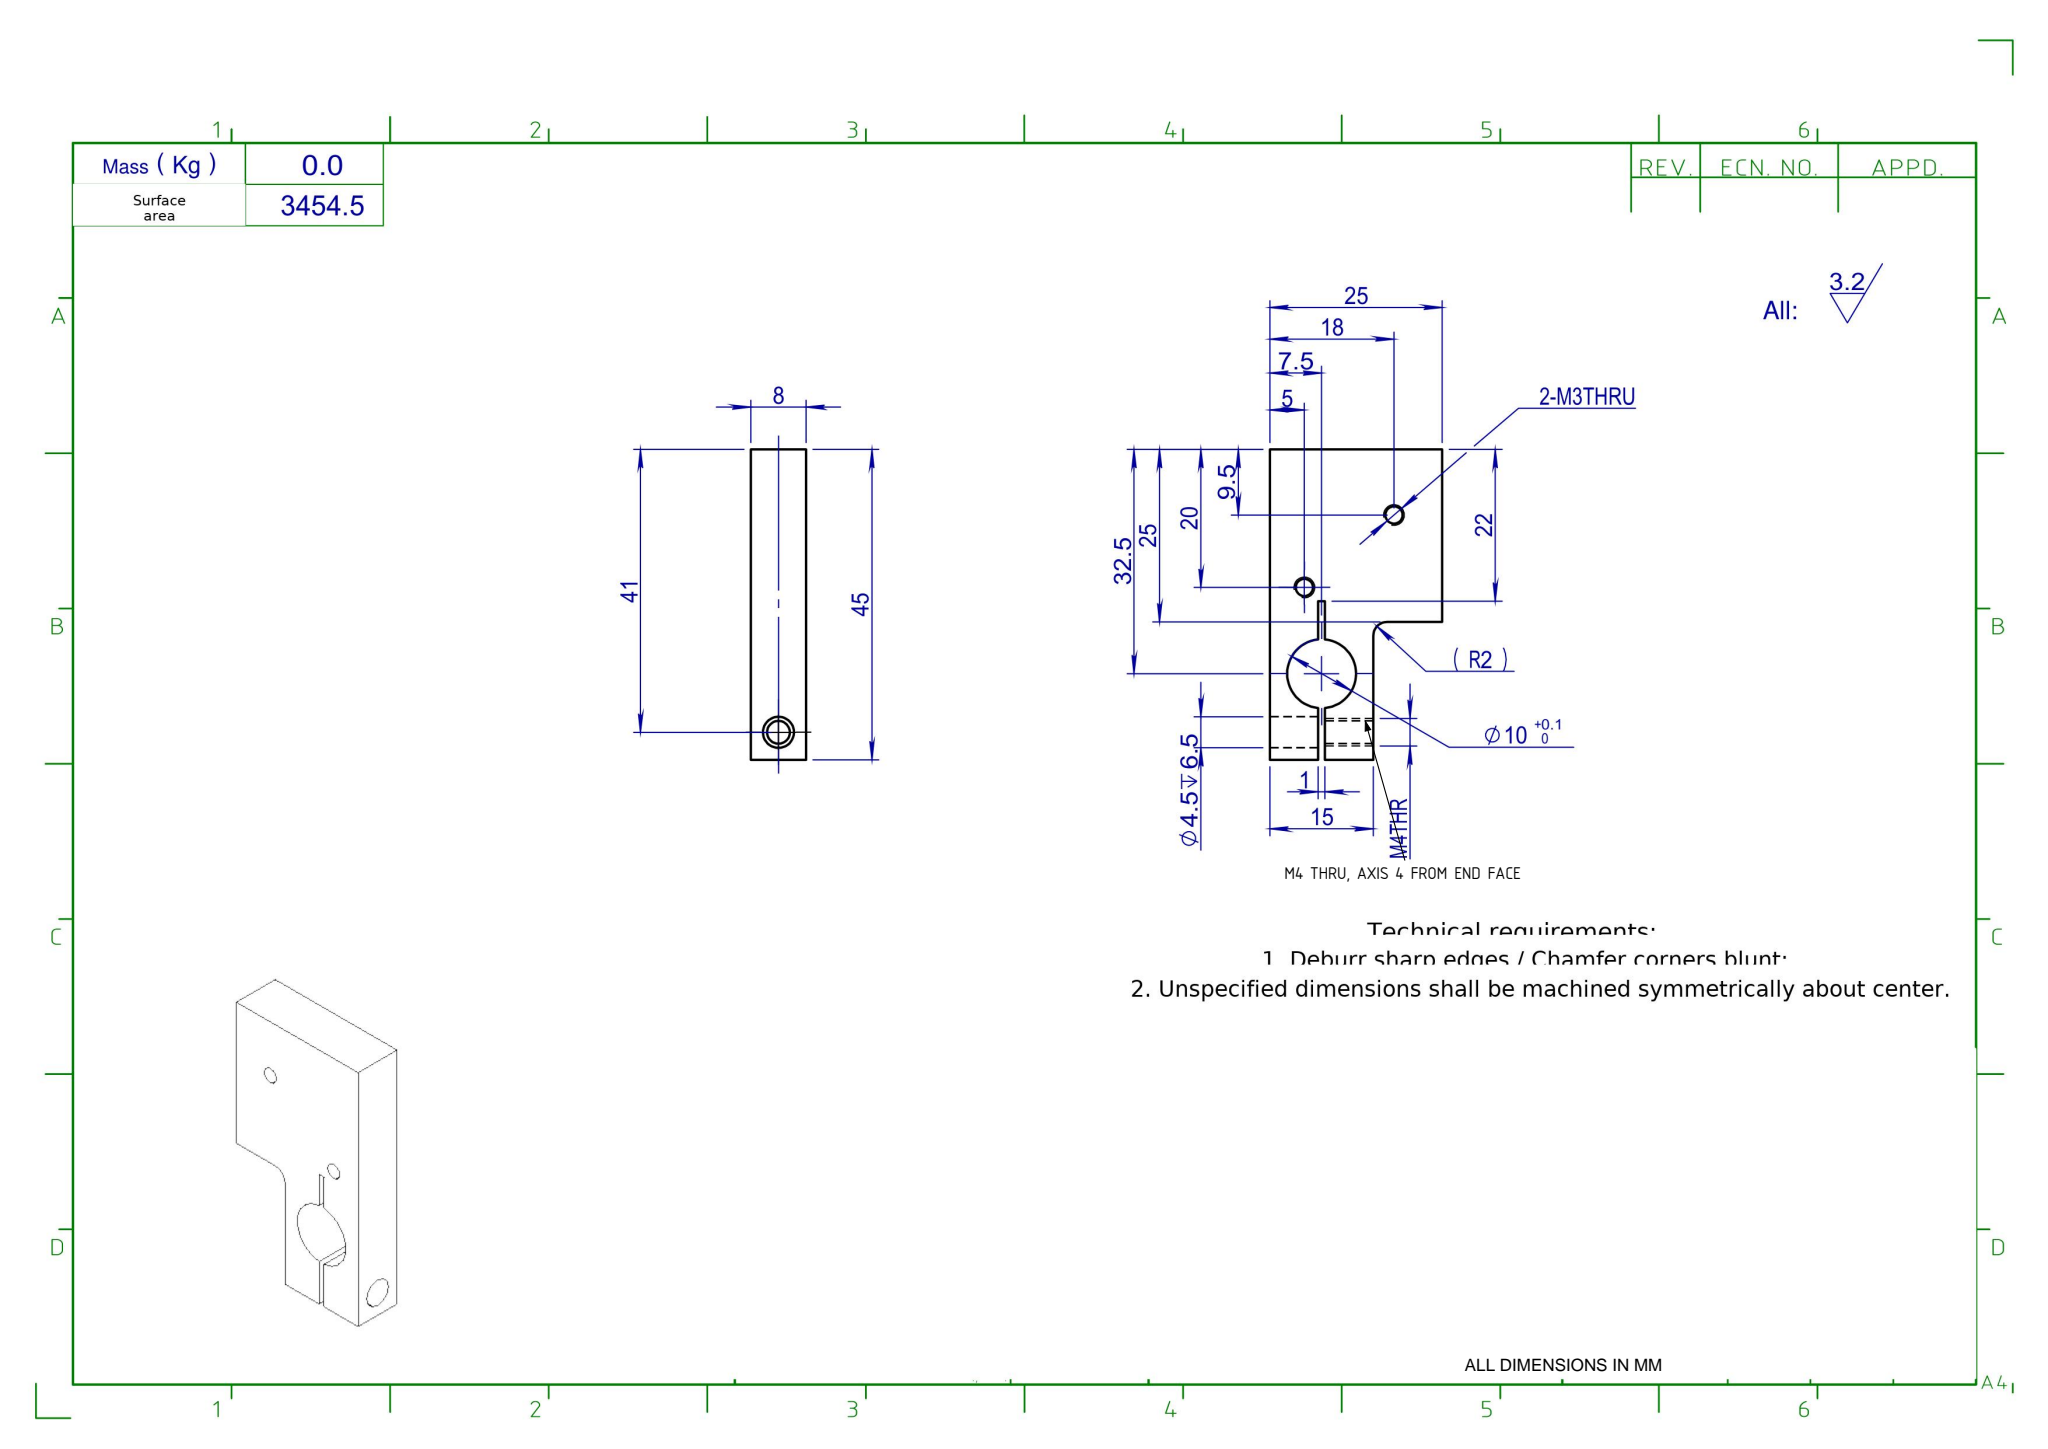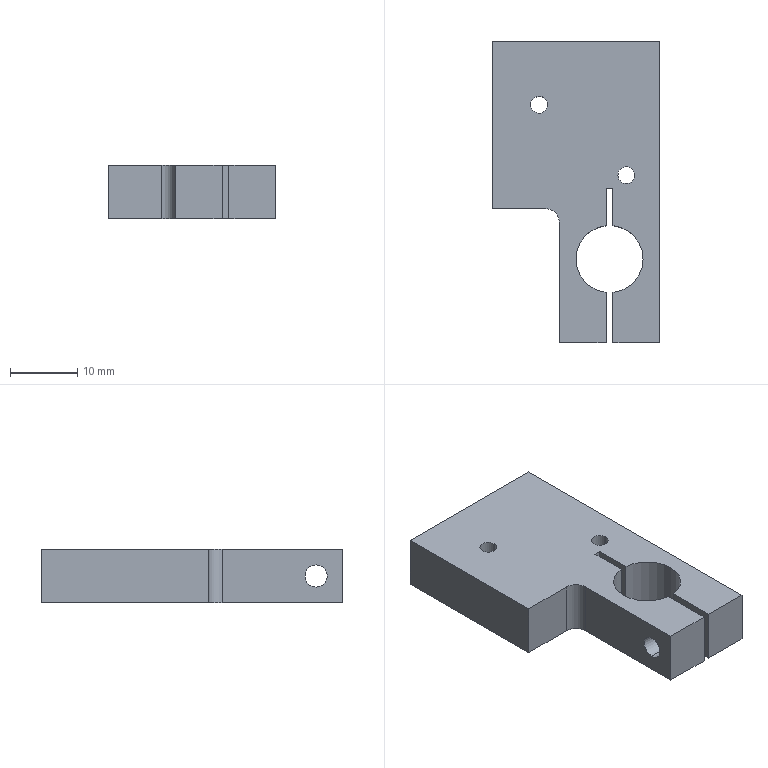Part | SolidWorks | mm | 1 solid | 26 faces | box 25 x 45 x 8 mm | volume 6425 mm3 | plane 14 | cylinder 12 | commonest cylinder face diameters 2.5 x4 10 x3 3.3 x2 4.5 x2 4 x1
Drawing notes:
M4 THRU 7 THK LEG (TAP DRILL Ø3.3), AXIS 4 FROM END FACE | from the solid: Cylinder dia 3.3, axis x, at y=4 z=4, from x=10 to x=17; leg faces x=10 and x=17 => 7 thru
build123d program:
from build123d import *

# Parameters (mm, degrees)
SKETCH1_W          = 15
SKETCH1_H          = 45
EXTRUDE1_DEPTH     = 8
SKETCH2_R          = 5
CUT_EXTRUDE1_DEPTH = 10
SKETCH3_W          = 1
SKETCH3_H          = 23
CUT_EXTRUDE2_DEPTH = 10
SKETCH8_W          = 8
SKETCH8_H          = 25
EXTRUDE2_DEPTH     = 10
SKETCH9_R          = 2.25
CUT_EXTRUDE3_DEPTH = 8
M4_TAPPED_HOLE1_D  = 3.3
M3_TAPPED_HOLE6_D  = 2.5
FILLET1_R          = 2


with BuildPart() as part:
    # Sketch1 → Extrude1 (new body)
    with BuildSketch(Plane.XY):
        with Locations((-14.432, 19.37)):
            Rectangle(SKETCH1_W, SKETCH1_H)
    extrude(amount=EXTRUDE1_DEPTH)

    # Sketch2 → Cut-Extrude1 (cut)
    with BuildSketch(Plane(origin=(0, 0, 0), x_dir=(-1, 0, 0), z_dir=(0, 0, -1))):
        with Locations((14.432, 9.37)):
            Circle(SKETCH2_R)
    extrude(amount=-CUT_EXTRUDE1_DEPTH, mode=Mode.SUBTRACT)

    # Sketch3 → Cut-Extrude2 (cut)
    with BuildSketch(Plane(origin=(0, 0, 0), x_dir=(-1, 0, 0), z_dir=(0, 0, -1))):
        with Locations((14.432, 8.37)):
            Rectangle(SKETCH3_W, SKETCH3_H)
    extrude(amount=-CUT_EXTRUDE2_DEPTH, mode=Mode.SUBTRACT)

    # Sketch8 → Extrude2 (add)
    with BuildSketch(Plane.ZY.offset(21.932)):
        with Locations((4, 29.37)):
            Rectangle(SKETCH8_W, SKETCH8_H)
    extrude(amount=EXTRUDE2_DEPTH)

    # Sketch9 → Cut-Extrude3 (cut)
    with BuildSketch(Plane.ZY.offset(6.932)):
        with Locations(Location((4, 0.8698, 0), (0, 0, 90))):
            Circle(SKETCH9_R)
    extrude(amount=CUT_EXTRUDE3_DEPTH, mode=Mode.SUBTRACT)

    # M4 Tapped Hole1 (through all)
    with Locations(Plane(origin=(-21.932, -5.228, 0.4606), x_dir=(0, 0, 1), z_dir=(-1, 0, 0))):
        with Locations((3.539, 6.098)):
            Hole(M4_TAPPED_HOLE1_D / 2)

    # M3 Tapped Hole6 (through all)
    with Locations(Plane(origin=(0, 0, 0), x_dir=(-1, 0, 0), z_dir=(0, 0, -1))):
        with Locations((11.932, 21.87), (24.932, 32.37)):
            Hole(M3_TAPPED_HOLE6_D / 2)

    # Fillet1
    fillet1_edges = [part.edges().sort_by_distance(p)[0] for p in [
        (-21.932, 16.87, 4),
    ]]
    fillet(fillet1_edges, radius=FILLET1_R)


solid = part.part
STEP:
#1=CARTESIAN_POINT('',(-13.182,21.87,8.));
#2=VERTEX_POINT('',#1);
#3=CARTESIAN_POINT('',(-10.682,21.87,8.));
#4=VERTEX_POINT('',#3);
#5=CARTESIAN_POINT('',(-11.932,21.87,8.));
#6=DIRECTION('',(0.,0.,1.));
#7=DIRECTION('',(1.,0.,0.));
#8=AXIS2_PLACEMENT_3D('',#5,#6,#7);
#9=CIRCLE('',#8,1.25);
#10=EDGE_CURVE('',#2,#4,#9,.T.);
#11=ORIENTED_EDGE('',*,*,#10,.T.);
#12=CARTESIAN_POINT('',(-10.682,21.87,-0.));
#13=VERTEX_POINT('',#12);
#14=CARTESIAN_POINT('',(-10.682,21.87,0.));
#15=DIRECTION('',(0.,0.,-1.));
#16=VECTOR('',#15,1000.);
#17=LINE('',#14,#16);
#18=EDGE_CURVE('',#4,#13,#17,.T.);
#19=ORIENTED_EDGE('',*,*,#18,.T.);
#20=CARTESIAN_POINT('',(-13.182,21.87,-0.));
#21=VERTEX_POINT('',#20);
#22=CARTESIAN_POINT('',(-11.932,21.87,-0.));
#23=DIRECTION('',(0.,0.,-1.));
#24=DIRECTION('',(-1.,0.,0.));
#25=AXIS2_PLACEMENT_3D('',#22,#23,#24);
#26=CIRCLE('',#25,1.25);
#27=EDGE_CURVE('',#13,#21,#26,.T.);
#28=ORIENTED_EDGE('',*,*,#27,.T.);
#29=CARTESIAN_POINT('',(-13.182,21.87,0.));
#30=DIRECTION('',(0.,0.,-1.));
#31=VECTOR('',#30,1000.);
#32=LINE('',#29,#31);
#33=EDGE_CURVE('',#2,#21,#32,.T.);
#34=ORIENTED_EDGE('',*,*,#33,.F.);
#35=EDGE_LOOP('',(#11,#19,#28,#34));
#36=FACE_OUTER_BOUND('',#35,.T.);
#37=CARTESIAN_POINT('',(-11.932,21.87,0.));
#38=DIRECTION('',(0.,0.,-1.));
#39=DIRECTION('',(-1.,0.,0.));
#40=AXIS2_PLACEMENT_3D('',#37,#38,#39);
#41=CYLINDRICAL_SURFACE('',#40,1.25);
#42=ADVANCED_FACE('',(#36),#41,.F.);
#43=CARTESIAN_POINT('',(-26.182,32.37,8.));
#44=VERTEX_POINT('',#43);
#45=CARTESIAN_POINT('',(-23.682,32.37,8.));
#46=VERTEX_POINT('',#45);
#47=CARTESIAN_POINT('',(-24.932,32.37,8.));
#48=DIRECTION('',(0.,0.,1.));
#49=DIRECTION('',(1.,0.,0.));
#50=AXIS2_PLACEMENT_3D('',#47,#48,#49);
#51=CIRCLE('',#50,1.25);
#52=EDGE_CURVE('',#44,#46,#51,.T.);
#53=ORIENTED_EDGE('',*,*,#52,.T.);
#54=CARTESIAN_POINT('',(-23.682,32.37,-0.));
#55=VERTEX_POINT('',#54);
#56=CARTESIAN_POINT('',(-23.682,32.37,0.));
#57=DIRECTION('',(0.,0.,-1.));
#58=VECTOR('',#57,1000.);
#59=LINE('',#56,#58);
#60=EDGE_CURVE('',#46,#55,#59,.T.);
#61=ORIENTED_EDGE('',*,*,#60,.T.);
#62=CARTESIAN_POINT('',(-26.182,32.37,-0.));
#63=VERTEX_POINT('',#62);
#64=CARTESIAN_POINT('',(-24.932,32.37,-0.));
#65=DIRECTION('',(0.,0.,-1.));
#66=DIRECTION('',(-1.,0.,0.));
#67=AXIS2_PLACEMENT_3D('',#64,#65,#66);
#68=CIRCLE('',#67,1.25);
#69=EDGE_CURVE('',#55,#63,#68,.T.);
#70=ORIENTED_EDGE('',*,*,#69,.T.);
#71=CARTESIAN_POINT('',(-26.182,32.37,0.));
#72=DIRECTION('',(0.,0.,-1.));
#73=VECTOR('',#72,1000.);
#74=LINE('',#71,#73);
#75=EDGE_CURVE('',#44,#63,#74,.T.);
#76=ORIENTED_EDGE('',*,*,#75,.F.);
#77=EDGE_LOOP('',(#53,#61,#70,#76));
#78=FACE_OUTER_BOUND('',#77,.T.);
#79=CARTESIAN_POINT('',(-24.932,32.37,0.));
#80=DIRECTION('',(0.,0.,-1.));
#81=DIRECTION('',(-1.,0.,0.));
#82=AXIS2_PLACEMENT_3D('',#79,#80,#81);
#83=CYLINDRICAL_SURFACE('',#82,1.25);
#84=ADVANCED_FACE('',(#78),#83,.F.);
#85=CARTESIAN_POINT('',(-14.932,0.8698,2.35));
#86=VERTEX_POINT('',#85);
#87=CARTESIAN_POINT('',(-14.932,0.8698,5.65));
#88=VERTEX_POINT('',#87);
#89=CARTESIAN_POINT('',(-14.932,0.8698,4.));
#90=DIRECTION('',(-1.,0.,0.));
#91=DIRECTION('',(0.,-1.,0.));
#92=AXIS2_PLACEMENT_3D('',#89,#90,#91);
#93=CIRCLE('',#92,1.65);
#94=EDGE_CURVE('',#86,#88,#93,.T.);
#95=ORIENTED_EDGE('',*,*,#94,.F.);
#96=CARTESIAN_POINT('',(-21.932,0.8698,2.35));
#97=VERTEX_POINT('',#96);
#98=CARTESIAN_POINT('',(-21.932,0.8698,2.35));
#99=DIRECTION('',(-1.,0.,0.));
#100=VECTOR('',#99,1000.);
#101=LINE('',#98,#100);
#102=EDGE_CURVE('',#86,#97,#101,.T.);
#103=ORIENTED_EDGE('',*,*,#102,.T.);
#104=CARTESIAN_POINT('',(-21.932,0.8698,5.65));
#105=VERTEX_POINT('',#104);
#106=CARTESIAN_POINT('',(-21.932,0.8698,4.));
#107=DIRECTION('',(-1.,0.,0.));
#108=DIRECTION('',(0.,0.,1.));
#109=AXIS2_PLACEMENT_3D('',#106,#107,#108);
#110=CIRCLE('',#109,1.65);
#111=EDGE_CURVE('',#97,#105,#110,.T.);
#112=ORIENTED_EDGE('',*,*,#111,.T.);
#113=CARTESIAN_POINT('',(-21.932,0.8698,5.65));
#114=DIRECTION('',(-1.,0.,0.));
#115=VECTOR('',#114,1000.);
#116=LINE('',#113,#115);
#117=EDGE_CURVE('',#88,#105,#116,.T.);
#118=ORIENTED_EDGE('',*,*,#117,.F.);
#119=EDGE_LOOP('',(#95,#103,#112,#118));
#120=FACE_OUTER_BOUND('',#119,.T.);
#121=CARTESIAN_POINT('',(-21.932,0.8698,4.));
#122=DIRECTION('',(-1.,0.,0.));
#123=DIRECTION('',(0.,0.,1.));
#124=AXIS2_PLACEMENT_3D('',#121,#122,#123);
#125=CYLINDRICAL_SURFACE('',#124,1.65);
#126=ADVANCED_FACE('',(#120),#125,.F.);
#127=CARTESIAN_POINT('',(-13.932,3.12,4.));
#128=VERTEX_POINT('',#127);
#129=CARTESIAN_POINT('',(-13.932,-1.38,4.));
#130=VERTEX_POINT('',#129);
#131=CARTESIAN_POINT('',(-13.932,0.8698,4.));
#132=DIRECTION('',(-1.,0.,0.));
#133=DIRECTION('',(0.,1.,0.));
#134=AXIS2_PLACEMENT_3D('',#131,#132,#133);
#135=CIRCLE('',#134,2.25);
#136=EDGE_CURVE('',#128,#130,#135,.T.);
#137=ORIENTED_EDGE('',*,*,#136,.T.);
#138=CARTESIAN_POINT('',(-6.932,-1.38,4.));
#139=VERTEX_POINT('',#138);
#140=CARTESIAN_POINT('',(-14.932,-1.38,4.));
#141=DIRECTION('',(1.,0.,0.));
#142=VECTOR('',#141,1000.);
#143=LINE('',#140,#142);
#144=EDGE_CURVE('',#130,#139,#143,.T.);
#145=ORIENTED_EDGE('',*,*,#144,.T.);
#146=CARTESIAN_POINT('',(-6.932,3.12,4.));
#147=VERTEX_POINT('',#146);
#148=CARTESIAN_POINT('',(-6.932,0.8698,4.));
#149=DIRECTION('',(-1.,-0.,0.));
#150=DIRECTION('',(0.,-1.,0.));
#151=AXIS2_PLACEMENT_3D('',#148,#149,#150);
#152=CIRCLE('',#151,2.25);
#153=EDGE_CURVE('',#147,#139,#152,.T.);
#154=ORIENTED_EDGE('',*,*,#153,.F.);
#155=CARTESIAN_POINT('',(-14.932,3.12,4.));
#156=DIRECTION('',(1.,0.,0.));
#157=VECTOR('',#156,1000.);
#158=LINE('',#155,#157);
#159=EDGE_CURVE('',#128,#147,#158,.T.);
#160=ORIENTED_EDGE('',*,*,#159,.F.);
#161=EDGE_LOOP('',(#137,#145,#154,#160));
#162=FACE_OUTER_BOUND('',#161,.T.);
#163=CARTESIAN_POINT('',(-14.932,0.8698,4.));
#164=DIRECTION('',(1.,0.,0.));
#165=DIRECTION('',(0.,1.,0.));
#166=AXIS2_PLACEMENT_3D('',#163,#164,#165);
#167=CYLINDRICAL_SURFACE('',#166,2.25);
#168=ADVANCED_FACE('',(#162),#167,.F.);
#169=CARTESIAN_POINT('',(-14.932,14.345,8.));
#170=VERTEX_POINT('',#169);
#171=CARTESIAN_POINT('',(-19.432,9.37,8.));
#172=VERTEX_POINT('',#171);
#173=CARTESIAN_POINT('',(-14.432,9.37,8.));
#174=DIRECTION('',(0.,0.,1.));
#175=DIRECTION('',(1.,0.,0.));
#176=AXIS2_PLACEMENT_3D('',#173,#174,#175);
#177=CIRCLE('',#176,5.);
#178=EDGE_CURVE('',#170,#172,#177,.T.);
#179=ORIENTED_EDGE('',*,*,#178,.T.);
#180=CARTESIAN_POINT('',(-19.432,9.37,0.));
#181=VERTEX_POINT('',#180);
#182=CARTESIAN_POINT('',(-19.432,9.37,10.));
#183=DIRECTION('',(0.,0.,-1.));
#184=VECTOR('',#183,1000.);
#185=LINE('',#182,#184);
#186=EDGE_CURVE('',#172,#181,#185,.T.);
#187=ORIENTED_EDGE('',*,*,#186,.T.);
#188=CARTESIAN_POINT('',(-14.932,14.345,0.));
#189=VERTEX_POINT('',#188);
#190=CARTESIAN_POINT('',(-14.432,9.37,0.));
#191=DIRECTION('',(0.,0.,-1.));
#192=DIRECTION('',(-1.,0.,0.));
#193=AXIS2_PLACEMENT_3D('',#190,#191,#192);
#194=CIRCLE('',#193,5.);
#195=EDGE_CURVE('',#181,#189,#194,.T.);
#196=ORIENTED_EDGE('',*,*,#195,.T.);
#197=CARTESIAN_POINT('',(-14.932,14.345,10.));
#198=DIRECTION('',(0.,0.,1.));
#199=VECTOR('',#198,1000.);
#200=LINE('',#197,#199);
#201=EDGE_CURVE('',#189,#170,#200,.T.);
#202=ORIENTED_EDGE('',*,*,#201,.T.);
#203=EDGE_LOOP('',(#179,#187,#196,#202));
#204=FACE_OUTER_BOUND('',#203,.T.);
#205=CARTESIAN_POINT('',(-14.432,9.37,10.));
#206=DIRECTION('',(0.,0.,-1.));
#207=DIRECTION('',(-1.,0.,0.));
#208=AXIS2_PLACEMENT_3D('',#205,#206,#207);
#209=CYLINDRICAL_SURFACE('',#208,5.);
#210=ADVANCED_FACE('',(#204),#209,.F.);
#211=CARTESIAN_POINT('',(-6.932,-3.13,0.));
#212=VERTEX_POINT('',#211);
#213=CARTESIAN_POINT('',(-6.932,41.87,0.));
#214=VERTEX_POINT('',#213);
#215=CARTESIAN_POINT('',(-6.932,41.87,0.));
#216=DIRECTION('',(-0.,1.,0.));
#217=VECTOR('',#216,1000.);
#218=LINE('',#215,#217);
#219=EDGE_CURVE('',#212,#214,#218,.T.);
#220=ORIENTED_EDGE('',*,*,#219,.T.);
#221=CARTESIAN_POINT('',(-6.932,41.87,8.));
#222=VERTEX_POINT('',#221);
#223=CARTESIAN_POINT('',(-6.932,41.87,8.));
#224=DIRECTION('',(0.,0.,-1.));
#225=VECTOR('',#224,1000.);
#226=LINE('',#223,#225);
#227=EDGE_CURVE('',#222,#214,#226,.T.);
#228=ORIENTED_EDGE('',*,*,#227,.F.);
#229=CARTESIAN_POINT('',(-6.932,-3.13,8.));
#230=VERTEX_POINT('',#229);
#231=CARTESIAN_POINT('',(-6.932,41.87,8.));
#232=DIRECTION('',(-0.,1.,0.));
#233=VECTOR('',#232,1000.);
#234=LINE('',#231,#233);
#235=EDGE_CURVE('',#230,#222,#234,.T.);
#236=ORIENTED_EDGE('',*,*,#235,.F.);
#237=CARTESIAN_POINT('',(-6.932,-3.13,8.));
#238=DIRECTION('',(0.,0.,-1.));
#239=VECTOR('',#238,1000.);
#240=LINE('',#237,#239);
#241=EDGE_CURVE('',#230,#212,#240,.T.);
#242=ORIENTED_EDGE('',*,*,#241,.T.);
#243=EDGE_LOOP('',(#220,#228,#236,#242));
#244=FACE_OUTER_BOUND('',#243,.T.);
#245=ORIENTED_EDGE('',*,*,#153,.T.);
#246=CARTESIAN_POINT('',(-6.932,0.8698,4.));
#247=DIRECTION('',(-1.,-0.,0.));
#248=DIRECTION('',(0.,-1.,0.));
#249=AXIS2_PLACEMENT_3D('',#246,#247,#248);
#250=CIRCLE('',#249,2.25);
#251=EDGE_CURVE('',#139,#147,#250,.T.);
#252=ORIENTED_EDGE('',*,*,#251,.T.);
#253=EDGE_LOOP('',(#245,#252));
#254=FACE_BOUND('',#253,.T.);
#255=CARTESIAN_POINT('',(-6.932,41.87,8.));
#256=DIRECTION('',(-1.,-0.,0.));
#257=DIRECTION('',(0.,-1.,0.));
#258=AXIS2_PLACEMENT_3D('',#255,#256,#257);
#259=PLANE('',#258);
#260=ADVANCED_FACE('',(#244,#254),#259,.F.);
#261=CARTESIAN_POINT('',(-13.932,-3.13,8.));
#262=VERTEX_POINT('',#261);
#263=CARTESIAN_POINT('',(-13.932,4.395,8.));
#264=VERTEX_POINT('',#263);
#265=CARTESIAN_POINT('',(-13.932,-3.13,8.));
#266=DIRECTION('',(0.,1.,0.));
#267=VECTOR('',#266,1000.);
#268=LINE('',#265,#267);
#269=EDGE_CURVE('',#262,#264,#268,.T.);
#270=ORIENTED_EDGE('',*,*,#269,.T.);
#271=CARTESIAN_POINT('',(-13.932,4.395,0.));
#272=VERTEX_POINT('',#271);
#273=CARTESIAN_POINT('',(-13.932,4.395,10.));
#274=DIRECTION('',(0.,0.,1.));
#275=VECTOR('',#274,1000.);
#276=LINE('',#273,#275);
#277=EDGE_CURVE('',#272,#264,#276,.T.);
#278=ORIENTED_EDGE('',*,*,#277,.F.);
#279=CARTESIAN_POINT('',(-13.932,-3.13,0.));
#280=VERTEX_POINT('',#279);
#281=CARTESIAN_POINT('',(-13.932,19.87,0.));
#282=DIRECTION('',(-0.,-1.,0.));
#283=VECTOR('',#282,1000.);
#284=LINE('',#281,#283);
#285=EDGE_CURVE('',#272,#280,#284,.T.);
#286=ORIENTED_EDGE('',*,*,#285,.T.);
#287=CARTESIAN_POINT('',(-13.932,-3.13,10.));
#288=DIRECTION('',(0.,0.,-1.));
#289=VECTOR('',#288,1000.);
#290=LINE('',#287,#289);
#291=EDGE_CURVE('',#262,#280,#290,.T.);
#292=ORIENTED_EDGE('',*,*,#291,.F.);
#293=EDGE_LOOP('',(#270,#278,#286,#292));
#294=FACE_OUTER_BOUND('',#293,.T.);
#295=ORIENTED_EDGE('',*,*,#136,.F.);
#296=CARTESIAN_POINT('',(-13.932,0.8698,4.));
#297=DIRECTION('',(-1.,0.,0.));
#298=DIRECTION('',(0.,1.,0.));
#299=AXIS2_PLACEMENT_3D('',#296,#297,#298);
#300=CIRCLE('',#299,2.25);
#301=EDGE_CURVE('',#130,#128,#300,.T.);
#302=ORIENTED_EDGE('',*,*,#301,.F.);
#303=EDGE_LOOP('',(#295,#302));
#304=FACE_BOUND('',#303,.T.);
#305=CARTESIAN_POINT('',(-13.932,19.87,10.));
#306=DIRECTION('',(1.,-0.,0.));
#307=DIRECTION('',(0.,1.,0.));
#308=AXIS2_PLACEMENT_3D('',#305,#306,#307);
#309=PLANE('',#308);
#310=ADVANCED_FACE('',(#294,#304),#309,.F.);
#311=CARTESIAN_POINT('',(-21.932,0.8698,4.));
#312=DIRECTION('',(-1.,0.,0.));
#313=DIRECTION('',(0.,0.,1.));
#314=AXIS2_PLACEMENT_3D('',#311,#312,#313);
#315=CIRCLE('',#314,1.65);
#316=EDGE_CURVE('',#105,#97,#315,.T.);
#317=ORIENTED_EDGE('',*,*,#316,.F.);
#318=ORIENTED_EDGE('',*,*,#111,.F.);
#319=EDGE_LOOP('',(#317,#318));
#320=FACE_BOUND('',#319,.T.);
#321=CARTESIAN_POINT('',(-21.932,14.87,8.));
#322=VERTEX_POINT('',#321);
#323=CARTESIAN_POINT('',(-21.932,-3.13,8.));
#324=VERTEX_POINT('',#323);
#325=CARTESIAN_POINT('',(-21.932,41.87,8.));
#326=DIRECTION('',(0.,-1.,0.));
#327=VECTOR('',#326,1000.);
#328=LINE('',#325,#327);
#329=EDGE_CURVE('',#322,#324,#328,.T.);
#330=ORIENTED_EDGE('',*,*,#329,.F.);
#331=CARTESIAN_POINT('',(-21.932,14.87,0.));
#332=VERTEX_POINT('',#331);
#333=CARTESIAN_POINT('',(-21.932,14.87,0.));
#334=DIRECTION('',(0.,0.,-1.));
#335=VECTOR('',#334,1000.);
#336=LINE('',#333,#335);
#337=EDGE_CURVE('',#322,#332,#336,.T.);
#338=ORIENTED_EDGE('',*,*,#337,.T.);
#339=CARTESIAN_POINT('',(-21.932,-3.13,0.));
#340=VERTEX_POINT('',#339);
#341=CARTESIAN_POINT('',(-21.932,41.87,0.));
#342=DIRECTION('',(0.,-1.,0.));
#343=VECTOR('',#342,1000.);
#344=LINE('',#341,#343);
#345=EDGE_CURVE('',#332,#340,#344,.T.);
#346=ORIENTED_EDGE('',*,*,#345,.T.);
#347=CARTESIAN_POINT('',(-21.932,-3.13,8.));
#348=DIRECTION('',(0.,0.,-1.));
#349=VECTOR('',#348,1000.);
#350=LINE('',#347,#349);
#351=EDGE_CURVE('',#324,#340,#350,.T.);
#352=ORIENTED_EDGE('',*,*,#351,.F.);
#353=EDGE_LOOP('',(#330,#338,#346,#352));
#354=FACE_OUTER_BOUND('',#353,.T.);
#355=CARTESIAN_POINT('',(-21.932,41.87,8.));
#356=DIRECTION('',(1.,0.,0.));
#357=DIRECTION('',(-0.,1.,0.));
#358=AXIS2_PLACEMENT_3D('',#355,#356,#357);
#359=PLANE('',#358);
#360=ADVANCED_FACE('',(#320,#354),#359,.F.);
#361=CARTESIAN_POINT('',(-21.932,-3.13,8.));
#362=DIRECTION('',(1.,0.,0.));
#363=VECTOR('',#362,1000.);
#364=LINE('',#361,#363);
#365=EDGE_CURVE('',#262,#230,#364,.T.);
#366=ORIENTED_EDGE('',*,*,#365,.F.);
#367=ORIENTED_EDGE('',*,*,#291,.T.);
#368=CARTESIAN_POINT('',(-21.932,-3.13,0.));
#369=DIRECTION('',(1.,0.,0.));
#370=VECTOR('',#369,1000.);
#371=LINE('',#368,#370);
#372=EDGE_CURVE('',#280,#212,#371,.T.);
#373=ORIENTED_EDGE('',*,*,#372,.T.);
#374=ORIENTED_EDGE('',*,*,#241,.F.);
#375=EDGE_LOOP('',(#366,#367,#373,#374));
#376=FACE_OUTER_BOUND('',#375,.T.);
#377=CARTESIAN_POINT('',(-21.932,-3.13,8.));
#378=DIRECTION('',(0.,1.,0.));
#379=DIRECTION('',(0.,0.,1.));
#380=AXIS2_PLACEMENT_3D('',#377,#378,#379);
#381=PLANE('',#380);
#382=ADVANCED_FACE('',(#376),#381,.F.);
#383=CARTESIAN_POINT('',(-13.932,14.345,0.));
#384=VERTEX_POINT('',#383);
#385=CARTESIAN_POINT('',(-14.432,9.37,0.));
#386=DIRECTION('',(0.,0.,-1.));
#387=DIRECTION('',(-1.,0.,0.));
#388=AXIS2_PLACEMENT_3D('',#385,#386,#387);
#389=CIRCLE('',#388,5.);
#390=EDGE_CURVE('',#384,#272,#389,.T.);
#391=ORIENTED_EDGE('',*,*,#390,.T.);
#392=ORIENTED_EDGE('',*,*,#277,.T.);
#393=CARTESIAN_POINT('',(-13.932,14.345,8.));
#394=VERTEX_POINT('',#393);
#395=CARTESIAN_POINT('',(-14.432,9.37,8.));
#396=DIRECTION('',(0.,0.,1.));
#397=DIRECTION('',(1.,0.,0.));
#398=AXIS2_PLACEMENT_3D('',#395,#396,#397);
#399=CIRCLE('',#398,5.);
#400=EDGE_CURVE('',#264,#394,#399,.T.);
#401=ORIENTED_EDGE('',*,*,#400,.T.);
#402=CARTESIAN_POINT('',(-13.932,14.345,10.));
#403=DIRECTION('',(0.,0.,-1.));
#404=VECTOR('',#403,1000.);
#405=LINE('',#402,#404);
#406=EDGE_CURVE('',#394,#384,#405,.T.);
#407=ORIENTED_EDGE('',*,*,#406,.T.);
#408=EDGE_LOOP('',(#391,#392,#401,#407));
#409=FACE_OUTER_BOUND('',#408,.T.);
#410=CARTESIAN_POINT('',(-14.432,9.37,10.));
#411=DIRECTION('',(0.,0.,-1.));
#412=DIRECTION('',(-1.,0.,0.));
#413=AXIS2_PLACEMENT_3D('',#410,#411,#412);
#414=CYLINDRICAL_SURFACE('',#413,5.);
#415=ADVANCED_FACE('',(#409),#414,.F.);
#416=CARTESIAN_POINT('',(-14.932,-3.13,0.));
#417=VERTEX_POINT('',#416);
#418=CARTESIAN_POINT('',(-21.932,-3.13,0.));
#419=DIRECTION('',(1.,0.,0.));
#420=VECTOR('',#419,1000.);
#421=LINE('',#418,#420);
#422=EDGE_CURVE('',#340,#417,#421,.T.);
#423=ORIENTED_EDGE('',*,*,#422,.T.);
#424=CARTESIAN_POINT('',(-14.932,-3.13,8.));
#425=VERTEX_POINT('',#424);
#426=CARTESIAN_POINT('',(-14.932,-3.13,10.));
#427=DIRECTION('',(0.,0.,-1.));
#428=VECTOR('',#427,1000.);
#429=LINE('',#426,#428);
#430=EDGE_CURVE('',#425,#417,#429,.T.);
#431=ORIENTED_EDGE('',*,*,#430,.F.);
#432=CARTESIAN_POINT('',(-21.932,-3.13,8.));
#433=DIRECTION('',(1.,0.,0.));
#434=VECTOR('',#433,1000.);
#435=LINE('',#432,#434);
#436=EDGE_CURVE('',#324,#425,#435,.T.);
#437=ORIENTED_EDGE('',*,*,#436,.F.);
#438=ORIENTED_EDGE('',*,*,#351,.T.);
#439=EDGE_LOOP('',(#423,#431,#437,#438));
#440=FACE_OUTER_BOUND('',#439,.T.);
#441=CARTESIAN_POINT('',(-21.932,-3.13,8.));
#442=DIRECTION('',(0.,1.,0.));
#443=DIRECTION('',(0.,0.,1.));
#444=AXIS2_PLACEMENT_3D('',#441,#442,#443);
#445=PLANE('',#444);
#446=ADVANCED_FACE('',(#440),#445,.F.);
#447=CARTESIAN_POINT('',(-31.932,41.87,0.));
#448=VERTEX_POINT('',#447);
#449=CARTESIAN_POINT('',(-21.932,41.87,0.));
#450=DIRECTION('',(-1.,0.,0.));
#451=VECTOR('',#450,1000.);
#452=LINE('',#449,#451);
#453=EDGE_CURVE('',#214,#448,#452,.T.);
#454=ORIENTED_EDGE('',*,*,#453,.T.);
#455=CARTESIAN_POINT('',(-31.932,41.87,8.));
#456=VERTEX_POINT('',#455);
#457=CARTESIAN_POINT('',(-31.932,41.87,0.));
#458=DIRECTION('',(0.,0.,-1.));
#459=VECTOR('',#458,1000.);
#460=LINE('',#457,#459);
#461=EDGE_CURVE('',#456,#448,#460,.T.);
#462=ORIENTED_EDGE('',*,*,#461,.F.);
#463=CARTESIAN_POINT('',(-21.932,41.87,8.));
#464=DIRECTION('',(-1.,0.,0.));
#465=VECTOR('',#464,1000.);
#466=LINE('',#463,#465);
#467=EDGE_CURVE('',#222,#456,#466,.T.);
#468=ORIENTED_EDGE('',*,*,#467,.F.);
#469=ORIENTED_EDGE('',*,*,#227,.T.);
#470=EDGE_LOOP('',(#454,#462,#468,#469));
#471=FACE_OUTER_BOUND('',#470,.T.);
#472=CARTESIAN_POINT('',(-21.932,41.87,8.));
#473=DIRECTION('',(0.,-1.,0.));
#474=DIRECTION('',(0.,0.,-1.));
#475=AXIS2_PLACEMENT_3D('',#472,#473,#474);
#476=PLANE('',#475);
#477=ADVANCED_FACE('',(#471),#476,.F.);
#478=ORIENTED_EDGE('',*,*,#10,.F.);
#479=CARTESIAN_POINT('',(-11.932,21.87,8.));
#480=DIRECTION('',(0.,0.,1.));
#481=DIRECTION('',(1.,0.,0.));
#482=AXIS2_PLACEMENT_3D('',#479,#480,#481);
#483=CIRCLE('',#482,1.25);
#484=EDGE_CURVE('',#4,#2,#483,.T.);
#485=ORIENTED_EDGE('',*,*,#484,.F.);
#486=EDGE_LOOP('',(#478,#485));
#487=FACE_BOUND('',#486,.T.);
#488=ORIENTED_EDGE('',*,*,#52,.F.);
#489=CARTESIAN_POINT('',(-24.932,32.37,8.));
#490=DIRECTION('',(0.,0.,1.));
#491=DIRECTION('',(1.,0.,0.));
#492=AXIS2_PLACEMENT_3D('',#489,#490,#491);
#493=CIRCLE('',#492,1.25);
#494=EDGE_CURVE('',#46,#44,#493,.T.);
#495=ORIENTED_EDGE('',*,*,#494,.F.);
#496=EDGE_LOOP('',(#488,#495));
#497=FACE_BOUND('',#496,.T.);
#498=ORIENTED_EDGE('',*,*,#269,.F.);
#499=ORIENTED_EDGE('',*,*,#365,.T.);
#500=ORIENTED_EDGE('',*,*,#235,.T.);
#501=ORIENTED_EDGE('',*,*,#467,.T.);
#502=CARTESIAN_POINT('',(-31.932,16.87,8.));
#503=VERTEX_POINT('',#502);
#504=CARTESIAN_POINT('',(-31.932,41.87,8.));
#505=DIRECTION('',(0.,1.,-0.));
#506=VECTOR('',#505,1000.);
#507=LINE('',#504,#506);
#508=EDGE_CURVE('',#503,#456,#507,.T.);
#509=ORIENTED_EDGE('',*,*,#508,.F.);
#510=CARTESIAN_POINT('',(-23.932,16.87,8.));
#511=VERTEX_POINT('',#510);
#512=CARTESIAN_POINT('',(-31.932,16.87,8.));
#513=DIRECTION('',(1.,0.,0.));
#514=VECTOR('',#513,1000.);
#515=LINE('',#512,#514);
#516=EDGE_CURVE('',#503,#511,#515,.T.);
#517=ORIENTED_EDGE('',*,*,#516,.T.);
#518=CARTESIAN_POINT('',(-23.932,14.87,8.));
#519=DIRECTION('',(0.,0.,-1.));
#520=DIRECTION('',(1.,-0.,0.));
#521=AXIS2_PLACEMENT_3D('',#518,#519,#520);
#522=CIRCLE('',#521,2.);
#523=EDGE_CURVE('',#511,#322,#522,.T.);
#524=ORIENTED_EDGE('',*,*,#523,.T.);
#525=ORIENTED_EDGE('',*,*,#329,.T.);
#526=ORIENTED_EDGE('',*,*,#436,.T.);
#527=CARTESIAN_POINT('',(-14.932,4.395,8.));
#528=VERTEX_POINT('',#527);
#529=CARTESIAN_POINT('',(-14.932,-3.13,8.));
#530=DIRECTION('',(-0.,-1.,0.));
#531=VECTOR('',#530,1000.);
#532=LINE('',#529,#531);
#533=EDGE_CURVE('',#528,#425,#532,.T.);
#534=ORIENTED_EDGE('',*,*,#533,.F.);
#535=CARTESIAN_POINT('',(-14.432,9.37,8.));
#536=DIRECTION('',(0.,0.,1.));
#537=DIRECTION('',(1.,0.,0.));
#538=AXIS2_PLACEMENT_3D('',#535,#536,#537);
#539=CIRCLE('',#538,5.);
#540=EDGE_CURVE('',#172,#528,#539,.T.);
#541=ORIENTED_EDGE('',*,*,#540,.F.);
#542=ORIENTED_EDGE('',*,*,#178,.F.);
#543=CARTESIAN_POINT('',(-14.932,19.87,8.));
#544=VERTEX_POINT('',#543);
#545=CARTESIAN_POINT('',(-14.932,-3.13,8.));
#546=DIRECTION('',(-0.,-1.,0.));
#547=VECTOR('',#546,1000.);
#548=LINE('',#545,#547);
#549=EDGE_CURVE('',#544,#170,#548,.T.);
#550=ORIENTED_EDGE('',*,*,#549,.F.);
#551=CARTESIAN_POINT('',(-13.932,19.87,8.));
#552=VERTEX_POINT('',#551);
#553=CARTESIAN_POINT('',(-21.932,19.87,8.));
#554=DIRECTION('',(-1.,0.,0.));
#555=VECTOR('',#554,1000.);
#556=LINE('',#553,#555);
#557=EDGE_CURVE('',#552,#544,#556,.T.);
#558=ORIENTED_EDGE('',*,*,#557,.F.);
#559=CARTESIAN_POINT('',(-13.932,-3.13,8.));
#560=DIRECTION('',(0.,1.,0.));
#561=VECTOR('',#560,1000.);
#562=LINE('',#559,#561);
#563=EDGE_CURVE('',#394,#552,#562,.T.);
#564=ORIENTED_EDGE('',*,*,#563,.F.);
#565=ORIENTED_EDGE('',*,*,#400,.F.);
#566=EDGE_LOOP('',(#498,#499,#500,#501,#509,#517,#524,#525,#526,#534,#541,#542,#550,#558,#564,#565));
#567=FACE_OUTER_BOUND('',#566,.T.);
#568=CARTESIAN_POINT('',(-21.932,-3.13,8.));
#569=DIRECTION('',(0.,0.,1.));
#570=DIRECTION('',(1.,0.,0.));
#571=AXIS2_PLACEMENT_3D('',#568,#569,#570);
#572=PLANE('',#571);
#573=ADVANCED_FACE('',(#487,#497,#567),#572,.T.);
#574=CARTESIAN_POINT('',(-11.932,21.87,-0.));
#575=DIRECTION('',(0.,0.,-1.));
#576=DIRECTION('',(-1.,0.,0.));
#577=AXIS2_PLACEMENT_3D('',#574,#575,#576);
#578=CIRCLE('',#577,1.25);
#579=EDGE_CURVE('',#21,#13,#578,.T.);
#580=ORIENTED_EDGE('',*,*,#579,.F.);
#581=ORIENTED_EDGE('',*,*,#27,.F.);
#582=EDGE_LOOP('',(#580,#581));
#583=FACE_BOUND('',#582,.T.);
#584=CARTESIAN_POINT('',(-24.932,32.37,-0.));
#585=DIRECTION('',(0.,0.,-1.));
#586=DIRECTION('',(-1.,0.,0.));
#587=AXIS2_PLACEMENT_3D('',#584,#585,#586);
#588=CIRCLE('',#587,1.25);
#589=EDGE_CURVE('',#63,#55,#588,.T.);
#590=ORIENTED_EDGE('',*,*,#589,.F.);
#591=ORIENTED_EDGE('',*,*,#69,.F.);
#592=EDGE_LOOP('',(#590,#591));
#593=FACE_BOUND('',#592,.T.);
#594=ORIENTED_EDGE('',*,*,#372,.F.);
#595=ORIENTED_EDGE('',*,*,#285,.F.);
#596=ORIENTED_EDGE('',*,*,#390,.F.);
#597=CARTESIAN_POINT('',(-13.932,19.87,0.));
#598=VERTEX_POINT('',#597);
#599=CARTESIAN_POINT('',(-13.932,19.87,0.));
#600=DIRECTION('',(-0.,-1.,0.));
#601=VECTOR('',#600,1000.);
#602=LINE('',#599,#601);
#603=EDGE_CURVE('',#598,#384,#602,.T.);
#604=ORIENTED_EDGE('',*,*,#603,.F.);
#605=CARTESIAN_POINT('',(-14.932,19.87,0.));
#606=VERTEX_POINT('',#605);
#607=CARTESIAN_POINT('',(-13.932,19.87,0.));
#608=DIRECTION('',(1.,0.,0.));
#609=VECTOR('',#608,1000.);
#610=LINE('',#607,#609);
#611=EDGE_CURVE('',#606,#598,#610,.T.);
#612=ORIENTED_EDGE('',*,*,#611,.F.);
#613=CARTESIAN_POINT('',(-14.932,19.87,0.));
#614=DIRECTION('',(0.,1.,0.));
#615=VECTOR('',#614,1000.);
#616=LINE('',#613,#615);
#617=EDGE_CURVE('',#189,#606,#616,.T.);
#618=ORIENTED_EDGE('',*,*,#617,.F.);
#619=ORIENTED_EDGE('',*,*,#195,.F.);
#620=CARTESIAN_POINT('',(-14.932,4.395,0.));
#621=VERTEX_POINT('',#620);
#622=CARTESIAN_POINT('',(-14.432,9.37,0.));
#623=DIRECTION('',(0.,0.,-1.));
#624=DIRECTION('',(-1.,0.,0.));
#625=AXIS2_PLACEMENT_3D('',#622,#623,#624);
#626=CIRCLE('',#625,5.);
#627=EDGE_CURVE('',#621,#181,#626,.T.);
#628=ORIENTED_EDGE('',*,*,#627,.F.);
#629=CARTESIAN_POINT('',(-14.932,19.87,0.));
#630=DIRECTION('',(0.,1.,0.));
#631=VECTOR('',#630,1000.);
#632=LINE('',#629,#631);
#633=EDGE_CURVE('',#417,#621,#632,.T.);
#634=ORIENTED_EDGE('',*,*,#633,.F.);
#635=ORIENTED_EDGE('',*,*,#422,.F.);
#636=ORIENTED_EDGE('',*,*,#345,.F.);
#637=CARTESIAN_POINT('',(-23.932,16.87,0.));
#638=VERTEX_POINT('',#637);
#639=CARTESIAN_POINT('',(-23.932,14.87,0.));
#640=DIRECTION('',(0.,0.,1.));
#641=DIRECTION('',(1.,0.,0.));
#642=AXIS2_PLACEMENT_3D('',#639,#640,#641);
#643=CIRCLE('',#642,2.);
#644=EDGE_CURVE('',#332,#638,#643,.T.);
#645=ORIENTED_EDGE('',*,*,#644,.T.);
#646=CARTESIAN_POINT('',(-31.932,16.87,0.));
#647=VERTEX_POINT('',#646);
#648=CARTESIAN_POINT('',(-31.932,16.87,0.));
#649=DIRECTION('',(1.,0.,0.));
#650=VECTOR('',#649,1000.);
#651=LINE('',#648,#650);
#652=EDGE_CURVE('',#647,#638,#651,.T.);
#653=ORIENTED_EDGE('',*,*,#652,.F.);
#654=CARTESIAN_POINT('',(-31.932,41.87,0.));
#655=DIRECTION('',(0.,-1.,0.));
#656=VECTOR('',#655,1000.);
#657=LINE('',#654,#656);
#658=EDGE_CURVE('',#448,#647,#657,.T.);
#659=ORIENTED_EDGE('',*,*,#658,.F.);
#660=ORIENTED_EDGE('',*,*,#453,.F.);
#661=ORIENTED_EDGE('',*,*,#219,.F.);
#662=EDGE_LOOP('',(#594,#595,#596,#604,#612,#618,#619,#628,#634,#635,#636,#645,#653,#659,#660,#661));
#663=FACE_OUTER_BOUND('',#662,.T.);
#664=CARTESIAN_POINT('',(-21.932,-3.13,0.));
#665=DIRECTION('',(0.,0.,1.));
#666=DIRECTION('',(1.,0.,0.));
#667=AXIS2_PLACEMENT_3D('',#664,#665,#666);
#668=PLANE('',#667);
#669=ADVANCED_FACE('',(#583,#593,#663),#668,.F.);
#670=ORIENTED_EDGE('',*,*,#186,.F.);
#671=ORIENTED_EDGE('',*,*,#540,.T.);
#672=CARTESIAN_POINT('',(-14.932,4.395,10.));
#673=DIRECTION('',(0.,0.,-1.));
#674=VECTOR('',#673,1000.);
#675=LINE('',#672,#674);
#676=EDGE_CURVE('',#528,#621,#675,.T.);
#677=ORIENTED_EDGE('',*,*,#676,.T.);
#678=ORIENTED_EDGE('',*,*,#627,.T.);
#679=EDGE_LOOP('',(#670,#671,#677,#678));
#680=FACE_OUTER_BOUND('',#679,.T.);
#681=CARTESIAN_POINT('',(-14.432,9.37,10.));
#682=DIRECTION('',(0.,0.,-1.));
#683=DIRECTION('',(-1.,0.,0.));
#684=AXIS2_PLACEMENT_3D('',#681,#682,#683);
#685=CYLINDRICAL_SURFACE('',#684,5.);
#686=ADVANCED_FACE('',(#680),#685,.F.);
#687=CARTESIAN_POINT('',(-14.932,0.8698,4.));
#688=DIRECTION('',(-1.,0.,0.));
#689=DIRECTION('',(0.,-1.,0.));
#690=AXIS2_PLACEMENT_3D('',#687,#688,#689);
#691=CIRCLE('',#690,1.65);
#692=EDGE_CURVE('',#88,#86,#691,.T.);
#693=ORIENTED_EDGE('',*,*,#692,.T.);
#694=ORIENTED_EDGE('',*,*,#94,.T.);
#695=EDGE_LOOP('',(#693,#694));
#696=FACE_BOUND('',#695,.T.);
#697=ORIENTED_EDGE('',*,*,#533,.T.);
#698=ORIENTED_EDGE('',*,*,#430,.T.);
#699=ORIENTED_EDGE('',*,*,#633,.T.);
#700=ORIENTED_EDGE('',*,*,#676,.F.);
#701=EDGE_LOOP('',(#697,#698,#699,#700));
#702=FACE_OUTER_BOUND('',#701,.T.);
#703=CARTESIAN_POINT('',(-14.932,19.87,10.));
#704=DIRECTION('',(-1.,0.,0.));
#705=DIRECTION('',(-0.,-1.,0.));
#706=AXIS2_PLACEMENT_3D('',#703,#704,#705);
#707=PLANE('',#706);
#708=ADVANCED_FACE('',(#696,#702),#707,.F.);
#709=ORIENTED_EDGE('',*,*,#549,.T.);
#710=ORIENTED_EDGE('',*,*,#201,.F.);
#711=ORIENTED_EDGE('',*,*,#617,.T.);
#712=CARTESIAN_POINT('',(-14.932,19.87,10.));
#713=DIRECTION('',(0.,0.,-1.));
#714=VECTOR('',#713,1000.);
#715=LINE('',#712,#714);
#716=EDGE_CURVE('',#544,#606,#715,.T.);
#717=ORIENTED_EDGE('',*,*,#716,.F.);
#718=EDGE_LOOP('',(#709,#710,#711,#717));
#719=FACE_OUTER_BOUND('',#718,.T.);
#720=CARTESIAN_POINT('',(-14.932,19.87,10.));
#721=DIRECTION('',(-1.,0.,0.));
#722=DIRECTION('',(-0.,-1.,0.));
#723=AXIS2_PLACEMENT_3D('',#720,#721,#722);
#724=PLANE('',#723);
#725=ADVANCED_FACE('',(#719),#724,.F.);
#726=ORIENTED_EDGE('',*,*,#563,.T.);
#727=CARTESIAN_POINT('',(-13.932,19.87,10.));
#728=DIRECTION('',(0.,0.,-1.));
#729=VECTOR('',#728,1000.);
#730=LINE('',#727,#729);
#731=EDGE_CURVE('',#552,#598,#730,.T.);
#732=ORIENTED_EDGE('',*,*,#731,.T.);
#733=ORIENTED_EDGE('',*,*,#603,.T.);
#734=ORIENTED_EDGE('',*,*,#406,.F.);
#735=EDGE_LOOP('',(#726,#732,#733,#734));
#736=FACE_OUTER_BOUND('',#735,.T.);
#737=CARTESIAN_POINT('',(-13.932,19.87,10.));
#738=DIRECTION('',(1.,-0.,0.));
#739=DIRECTION('',(0.,1.,0.));
#740=AXIS2_PLACEMENT_3D('',#737,#738,#739);
#741=PLANE('',#740);
#742=ADVANCED_FACE('',(#736),#741,.F.);
#743=ORIENTED_EDGE('',*,*,#557,.T.);
#744=ORIENTED_EDGE('',*,*,#716,.T.);
#745=ORIENTED_EDGE('',*,*,#611,.T.);
#746=ORIENTED_EDGE('',*,*,#731,.F.);
#747=EDGE_LOOP('',(#743,#744,#745,#746));
#748=FACE_OUTER_BOUND('',#747,.T.);
#749=CARTESIAN_POINT('',(-13.932,19.87,10.));
#750=DIRECTION('',(0.,1.,0.));
#751=DIRECTION('',(0.,0.,1.));
#752=AXIS2_PLACEMENT_3D('',#749,#750,#751);
#753=PLANE('',#752);
#754=ADVANCED_FACE('',(#748),#753,.F.);
#755=ORIENTED_EDGE('',*,*,#652,.T.);
#756=CARTESIAN_POINT('',(-23.932,16.87,8.));
#757=DIRECTION('',(0.,0.,1.));
#758=VECTOR('',#757,1000.);
#759=LINE('',#756,#758);
#760=EDGE_CURVE('',#638,#511,#759,.T.);
#761=ORIENTED_EDGE('',*,*,#760,.T.);
#762=ORIENTED_EDGE('',*,*,#516,.F.);
#763=CARTESIAN_POINT('',(-31.932,16.87,0.));
#764=DIRECTION('',(0.,0.,1.));
#765=VECTOR('',#764,1000.);
#766=LINE('',#763,#765);
#767=EDGE_CURVE('',#647,#503,#766,.T.);
#768=ORIENTED_EDGE('',*,*,#767,.F.);
#769=EDGE_LOOP('',(#755,#761,#762,#768));
#770=FACE_OUTER_BOUND('',#769,.T.);
#771=CARTESIAN_POINT('',(-31.932,16.87,0.));
#772=DIRECTION('',(0.,1.,0.));
#773=DIRECTION('',(0.,0.,1.));
#774=AXIS2_PLACEMENT_3D('',#771,#772,#773);
#775=PLANE('',#774);
#776=ADVANCED_FACE('',(#770),#775,.F.);
#777=ORIENTED_EDGE('',*,*,#658,.T.);
#778=ORIENTED_EDGE('',*,*,#767,.T.);
#779=ORIENTED_EDGE('',*,*,#508,.T.);
#780=ORIENTED_EDGE('',*,*,#461,.T.);
#781=EDGE_LOOP('',(#777,#778,#779,#780));
#782=FACE_OUTER_BOUND('',#781,.T.);
#783=CARTESIAN_POINT('',(-31.932,16.87,0.));
#784=DIRECTION('',(-1.,0.,0.));
#785=DIRECTION('',(0.,0.,1.));
#786=AXIS2_PLACEMENT_3D('',#783,#784,#785);
#787=PLANE('',#786);
#788=ADVANCED_FACE('',(#782),#787,.T.);
#789=ORIENTED_EDGE('',*,*,#144,.F.);
#790=ORIENTED_EDGE('',*,*,#301,.T.);
#791=ORIENTED_EDGE('',*,*,#159,.T.);
#792=ORIENTED_EDGE('',*,*,#251,.F.);
#793=EDGE_LOOP('',(#789,#790,#791,#792));
#794=FACE_OUTER_BOUND('',#793,.T.);
#795=CARTESIAN_POINT('',(-14.932,0.8698,4.));
#796=DIRECTION('',(1.,0.,0.));
#797=DIRECTION('',(0.,1.,0.));
#798=AXIS2_PLACEMENT_3D('',#795,#796,#797);
#799=CYLINDRICAL_SURFACE('',#798,2.25);
#800=ADVANCED_FACE('',(#794),#799,.F.);
#801=ORIENTED_EDGE('',*,*,#102,.F.);
#802=ORIENTED_EDGE('',*,*,#692,.F.);
#803=ORIENTED_EDGE('',*,*,#117,.T.);
#804=ORIENTED_EDGE('',*,*,#316,.T.);
#805=EDGE_LOOP('',(#801,#802,#803,#804));
#806=FACE_OUTER_BOUND('',#805,.T.);
#807=CARTESIAN_POINT('',(-21.932,0.8698,4.));
#808=DIRECTION('',(-1.,0.,0.));
#809=DIRECTION('',(0.,0.,1.));
#810=AXIS2_PLACEMENT_3D('',#807,#808,#809);
#811=CYLINDRICAL_SURFACE('',#810,1.65);
#812=ADVANCED_FACE('',(#806),#811,.F.);
#813=ORIENTED_EDGE('',*,*,#60,.F.);
#814=ORIENTED_EDGE('',*,*,#494,.T.);
#815=ORIENTED_EDGE('',*,*,#75,.T.);
#816=ORIENTED_EDGE('',*,*,#589,.T.);
#817=EDGE_LOOP('',(#813,#814,#815,#816));
#818=FACE_OUTER_BOUND('',#817,.T.);
#819=CARTESIAN_POINT('',(-24.932,32.37,0.));
#820=DIRECTION('',(0.,0.,-1.));
#821=DIRECTION('',(-1.,0.,0.));
#822=AXIS2_PLACEMENT_3D('',#819,#820,#821);
#823=CYLINDRICAL_SURFACE('',#822,1.25);
#824=ADVANCED_FACE('',(#818),#823,.F.);
#825=ORIENTED_EDGE('',*,*,#18,.F.);
#826=ORIENTED_EDGE('',*,*,#484,.T.);
#827=ORIENTED_EDGE('',*,*,#33,.T.);
#828=ORIENTED_EDGE('',*,*,#579,.T.);
#829=EDGE_LOOP('',(#825,#826,#827,#828));
#830=FACE_OUTER_BOUND('',#829,.T.);
#831=CARTESIAN_POINT('',(-11.932,21.87,0.));
#832=DIRECTION('',(0.,0.,-1.));
#833=DIRECTION('',(-1.,0.,0.));
#834=AXIS2_PLACEMENT_3D('',#831,#832,#833);
#835=CYLINDRICAL_SURFACE('',#834,1.25);
#836=ADVANCED_FACE('',(#830),#835,.F.);
#837=ORIENTED_EDGE('',*,*,#644,.F.);
#838=ORIENTED_EDGE('',*,*,#337,.F.);
#839=ORIENTED_EDGE('',*,*,#523,.F.);
#840=ORIENTED_EDGE('',*,*,#760,.F.);
#841=EDGE_LOOP('',(#837,#838,#839,#840));
#842=FACE_OUTER_BOUND('',#841,.T.);
#843=CARTESIAN_POINT('',(-23.932,14.87,0.));
#844=DIRECTION('',(0.,0.,-1.));
#845=DIRECTION('',(-1.,0.,0.));
#846=AXIS2_PLACEMENT_3D('',#843,#844,#845);
#847=CYLINDRICAL_SURFACE('',#846,2.);
#848=ADVANCED_FACE('',(#842),#847,.F.);
#849=CLOSED_SHELL('',(#42,#84,#126,#168,#210,#260,#310,#360,#382,#415,#446,#477,#573,#669,#686,#708,#725,#742,#754,#776,#788,#800,#812,#824,#836,#848));
#850=MANIFOLD_SOLID_BREP('',#849);
#851=CARTESIAN_POINT('',(0.,0.,0.));
#852=DIRECTION('',(0.,0.,1.));
#853=DIRECTION('',(1.,0.,0.));
#854=AXIS2_PLACEMENT_3D('',#851,#852,#853);
#855=(LENGTH_UNIT()NAMED_UNIT(*)SI_UNIT(.MILLI.,.METRE.));
#856=UNCERTAINTY_MEASURE_WITH_UNIT(LENGTH_MEASURE(0.00001),#855,'','');
#857=(NAMED_UNIT(*)PLANE_ANGLE_UNIT()SI_UNIT($,.RADIAN.));
#858=(NAMED_UNIT(*)SI_UNIT($,.STERADIAN.)SOLID_ANGLE_UNIT());
#859=(GEOMETRIC_REPRESENTATION_CONTEXT(3)GLOBAL_UNCERTAINTY_ASSIGNED_CONTEXT((#856))GLOBAL_UNIT_ASSIGNED_CONTEXT((#855,#857,#858))REPRESENTATION_CONTEXT('',''));
#860=ADVANCED_BREP_SHAPE_REPRESENTATION('',(#850,#854),#859);